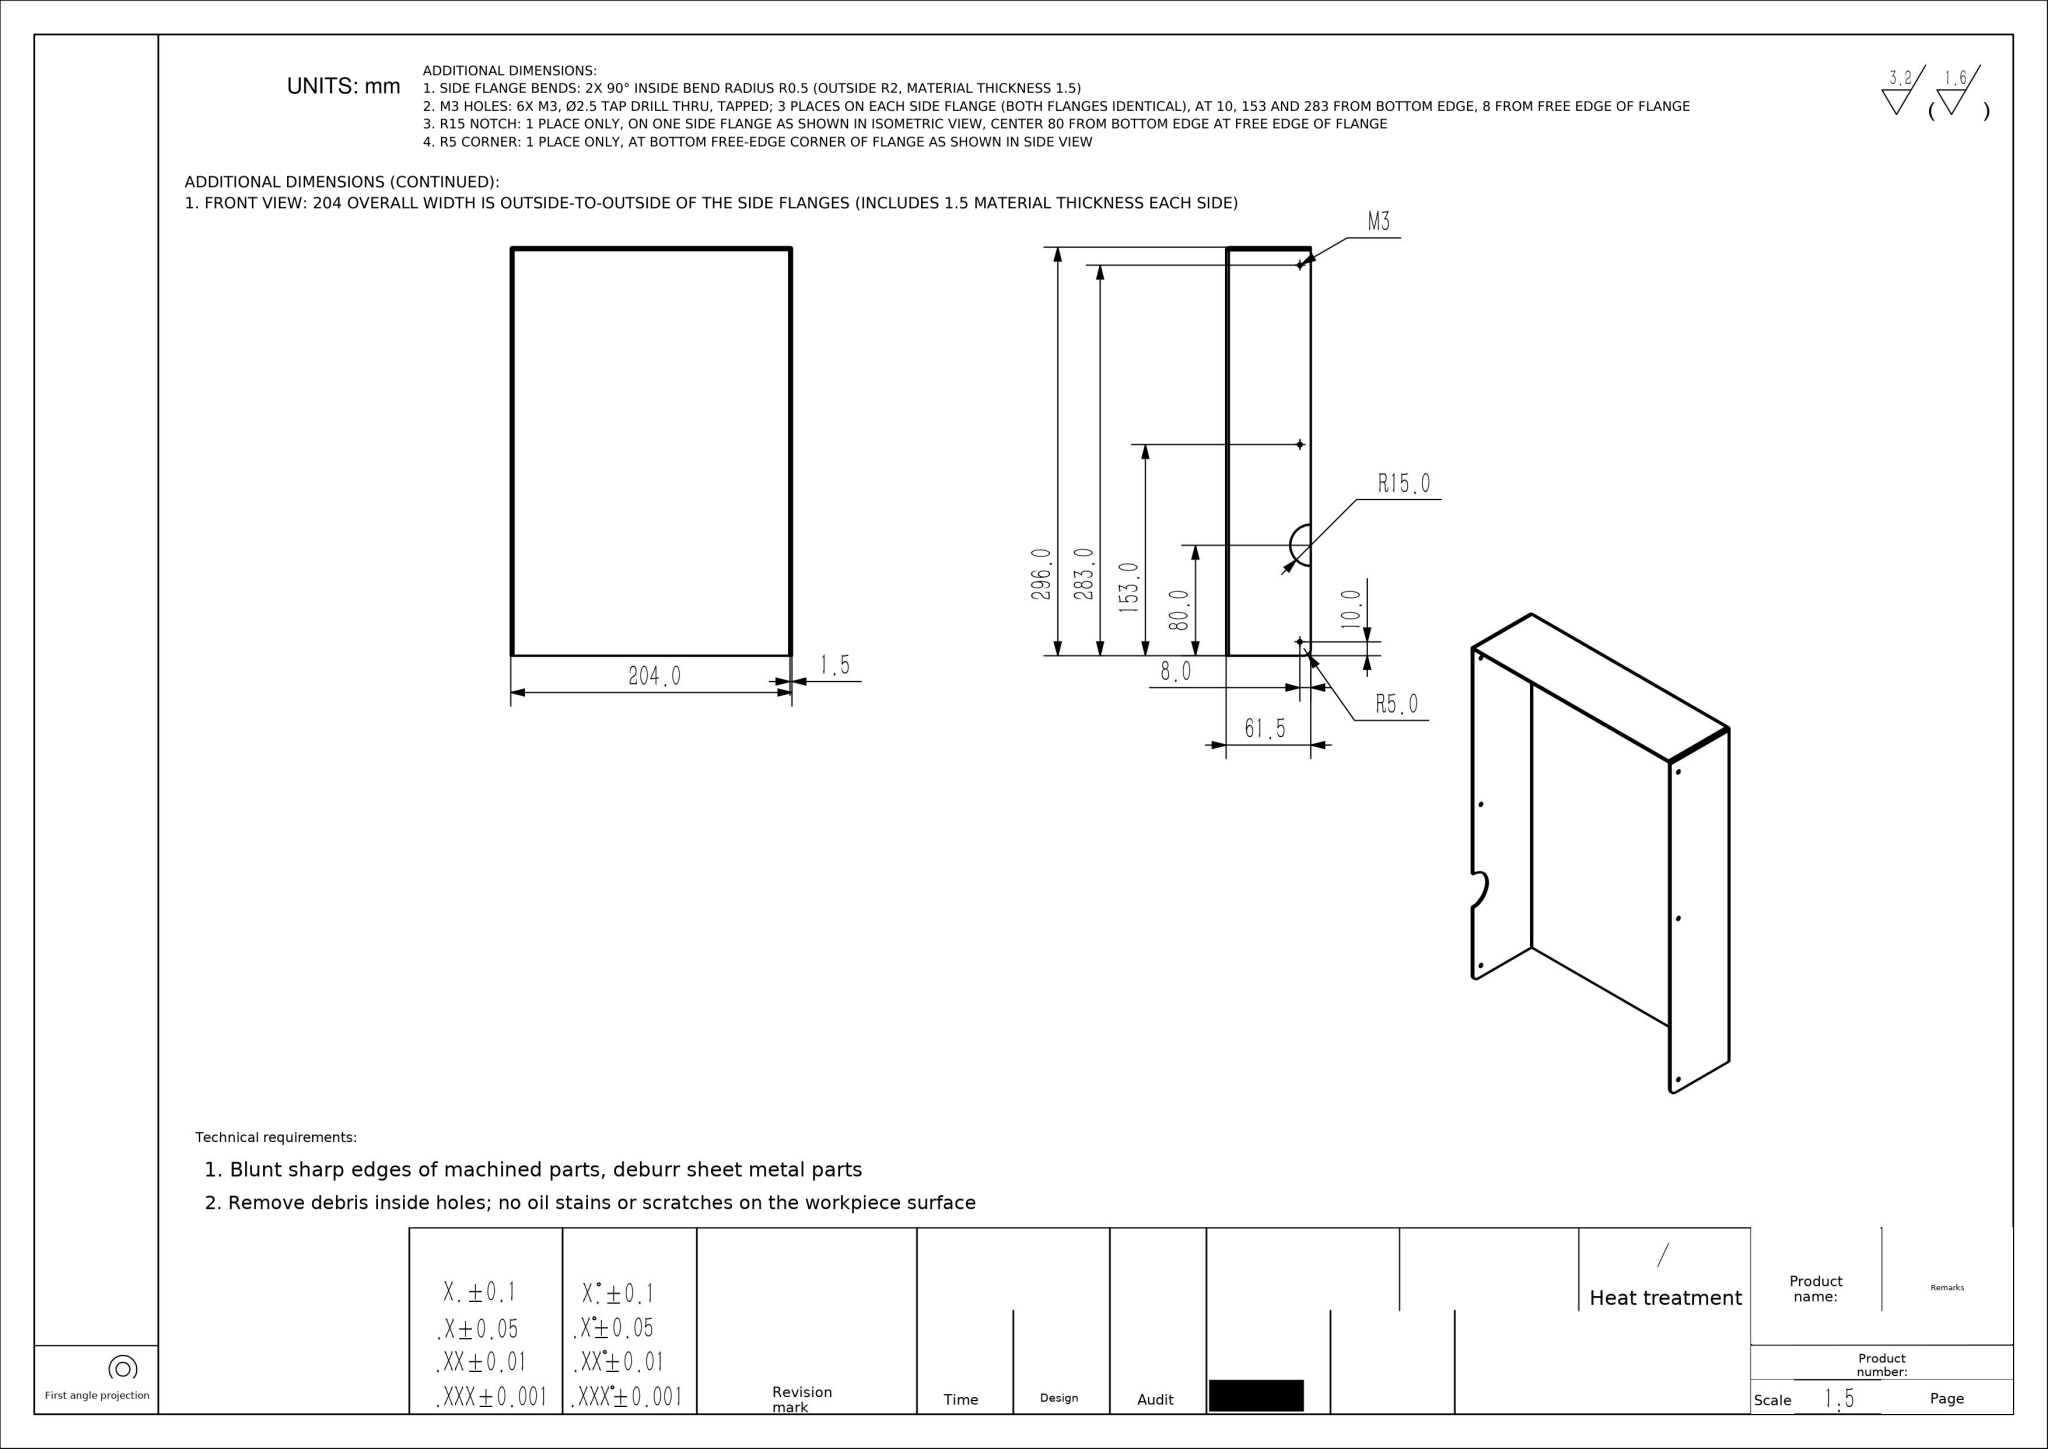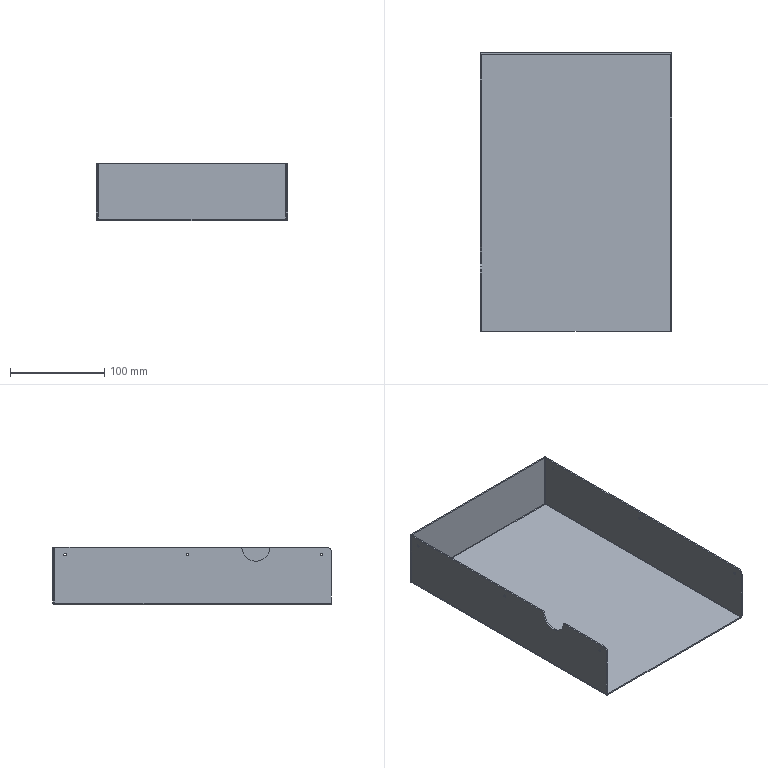Part | NX | mm | 1 solid | 60 faces | box 204 x 296 x 61.5 mm | volume 160690 mm3 | plane 27 | cylinder 23 | spline 10 | commonest cylinder face diameters 2.5 x12 4 x3 1 x3 2 x2 10 x2 30 x1